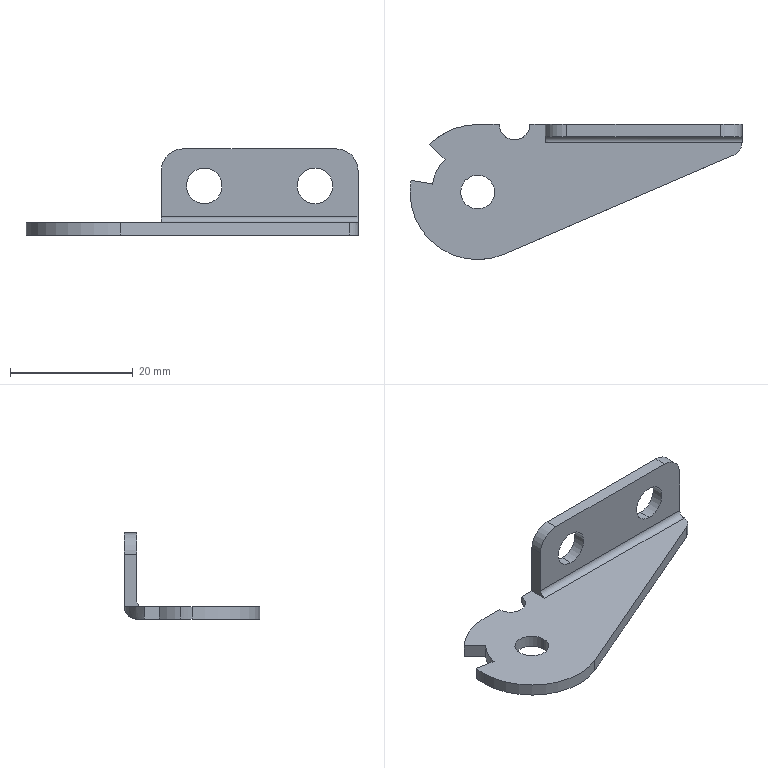Component | SolidWorks | MHPUS204-38-33-A-1_34-1 | 1 solid | 27 faces | box 54 x 22 x 14 mm | volume 2071 mm3 | cylinder 17 | plane 10 | commonest cylinder face diameters 5.8 x4 22 x3 5.5 x2 4 x2 7 x2 5 x1 4.4 x1 15 x1
STEP:
#1=CARTESIAN_POINT('',(20.81,-0.9055,1.98));
#2=VERTEX_POINT('',#1);
#3=CARTESIAN_POINT('',(20.594,-0.9055,1.98));
#4=VERTEX_POINT('',#3);
#5=CARTESIAN_POINT('',(20.702,-0.9055,1.98));
#6=DIRECTION('',(0.,0.,-1.));
#7=DIRECTION('',(-1.,0.,0.));
#8=AXIS2_PLACEMENT_3D('',#5,#6,#7);
#9=CIRCLE('',#8,0.1083);
#10=EDGE_CURVE('',#2,#4,#9,.T.);
#11=ORIENTED_EDGE('',*,*,#10,.F.);
#12=CARTESIAN_POINT('',(20.81,-0.9055,1.902));
#13=VERTEX_POINT('',#12);
#14=CARTESIAN_POINT('',(20.81,-0.9055,1.902));
#15=DIRECTION('',(0.,0.,-1.));
#16=VECTOR('',#15,39.37);
#17=LINE('',#14,#16);
#18=EDGE_CURVE('',#2,#13,#17,.T.);
#19=ORIENTED_EDGE('',*,*,#18,.T.);
#20=CARTESIAN_POINT('',(20.594,-0.9055,1.902));
#21=VERTEX_POINT('',#20);
#22=CARTESIAN_POINT('',(20.702,-0.9055,1.902));
#23=DIRECTION('',(0.,0.,-1.));
#24=DIRECTION('',(-1.,0.,0.));
#25=AXIS2_PLACEMENT_3D('',#22,#23,#24);
#26=CIRCLE('',#25,0.1083);
#27=EDGE_CURVE('',#13,#21,#26,.T.);
#28=ORIENTED_EDGE('',*,*,#27,.T.);
#29=CARTESIAN_POINT('',(20.594,-0.9055,1.902));
#30=DIRECTION('',(0.,0.,-1.));
#31=VECTOR('',#30,39.37);
#32=LINE('',#29,#31);
#33=EDGE_CURVE('',#4,#21,#32,.T.);
#34=ORIENTED_EDGE('',*,*,#33,.F.);
#35=EDGE_LOOP('',(#11,#19,#28,#34));
#36=FACE_OUTER_BOUND('',#35,.T.);
#37=CARTESIAN_POINT('',(20.702,-0.9055,1.902));
#38=DIRECTION('',(0.,0.,-1.));
#39=DIRECTION('',(-1.,0.,0.));
#40=AXIS2_PLACEMENT_3D('',#37,#38,#39);
#41=CYLINDRICAL_SURFACE('',#40,0.1083);
#42=ADVANCED_FACE('',(#36),#41,.F.);
#43=CARTESIAN_POINT('',(20.874,-1.303,1.98));
#44=VERTEX_POINT('',#43);
#45=CARTESIAN_POINT('',(20.269,-0.9055,1.98));
#46=VERTEX_POINT('',#45);
#47=CARTESIAN_POINT('',(20.702,-0.9055,1.98));
#48=DIRECTION('',(0.,0.,-1.));
#49=DIRECTION('',(-1.,0.,0.));
#50=AXIS2_PLACEMENT_3D('',#47,#48,#49);
#51=CIRCLE('',#50,0.4331);
#52=EDGE_CURVE('',#44,#46,#51,.T.);
#53=ORIENTED_EDGE('',*,*,#52,.T.);
#54=CARTESIAN_POINT('',(20.269,-0.9055,1.902));
#55=VERTEX_POINT('',#54);
#56=CARTESIAN_POINT('',(20.269,-0.9055,1.902));
#57=DIRECTION('',(0.,0.,-1.));
#58=VECTOR('',#57,39.37);
#59=LINE('',#56,#58);
#60=EDGE_CURVE('',#46,#55,#59,.T.);
#61=ORIENTED_EDGE('',*,*,#60,.T.);
#62=CARTESIAN_POINT('',(20.874,-1.303,1.902));
#63=VERTEX_POINT('',#62);
#64=CARTESIAN_POINT('',(20.702,-0.9055,1.902));
#65=DIRECTION('',(0.,0.,1.));
#66=DIRECTION('',(-1.,0.,0.));
#67=AXIS2_PLACEMENT_3D('',#64,#65,#66);
#68=CIRCLE('',#67,0.4331);
#69=EDGE_CURVE('',#55,#63,#68,.T.);
#70=ORIENTED_EDGE('',*,*,#69,.T.);
#71=CARTESIAN_POINT('',(20.874,-1.303,1.902));
#72=DIRECTION('',(0.,0.,-1.));
#73=VECTOR('',#72,39.37);
#74=LINE('',#71,#73);
#75=EDGE_CURVE('',#44,#63,#74,.T.);
#76=ORIENTED_EDGE('',*,*,#75,.F.);
#77=EDGE_LOOP('',(#53,#61,#70,#76));
#78=FACE_OUTER_BOUND('',#77,.T.);
#79=CARTESIAN_POINT('',(20.702,-0.9055,1.902));
#80=DIRECTION('',(0.,0.,-1.));
#81=DIRECTION('',(-1.,0.,0.));
#82=AXIS2_PLACEMENT_3D('',#79,#80,#81);
#83=CYLINDRICAL_SURFACE('',#82,0.4331);
#84=ADVANCED_FACE('',(#78),#83,.T.);
#85=CARTESIAN_POINT('',(21.411,-0.5512,2.331));
#86=VERTEX_POINT('',#85);
#87=CARTESIAN_POINT('',(21.411,-0.5512,2.102));
#88=VERTEX_POINT('',#87);
#89=CARTESIAN_POINT('',(21.411,-0.5512,2.217));
#90=DIRECTION('',(0.,-1.,0.));
#91=DIRECTION('',(0.,0.,1.));
#92=AXIS2_PLACEMENT_3D('',#89,#90,#91);
#93=CIRCLE('',#92,0.1142);
#94=EDGE_CURVE('',#86,#88,#93,.T.);
#95=ORIENTED_EDGE('',*,*,#94,.T.);
#96=CARTESIAN_POINT('',(21.411,-0.4724,2.102));
#97=VERTEX_POINT('',#96);
#98=CARTESIAN_POINT('',(21.411,-0.3937,2.102));
#99=DIRECTION('',(0.,1.,0.));
#100=VECTOR('',#99,39.37);
#101=LINE('',#98,#100);
#102=EDGE_CURVE('',#88,#97,#101,.T.);
#103=ORIENTED_EDGE('',*,*,#102,.T.);
#104=CARTESIAN_POINT('',(21.411,-0.4724,2.331));
#105=VERTEX_POINT('',#104);
#106=CARTESIAN_POINT('',(21.411,-0.4724,2.217));
#107=DIRECTION('',(0.,-1.,0.));
#108=DIRECTION('',(0.,0.,1.));
#109=AXIS2_PLACEMENT_3D('',#106,#107,#108);
#110=CIRCLE('',#109,0.1142);
#111=EDGE_CURVE('',#105,#97,#110,.T.);
#112=ORIENTED_EDGE('',*,*,#111,.F.);
#113=CARTESIAN_POINT('',(21.411,-0.3937,2.331));
#114=DIRECTION('',(0.,1.,0.));
#115=VECTOR('',#114,39.37);
#116=LINE('',#113,#115);
#117=EDGE_CURVE('',#86,#105,#116,.T.);
#118=ORIENTED_EDGE('',*,*,#117,.F.);
#119=EDGE_LOOP('',(#95,#103,#112,#118));
#120=FACE_OUTER_BOUND('',#119,.T.);
#121=CARTESIAN_POINT('',(21.411,-0.3937,2.217));
#122=DIRECTION('',(0.,1.,0.));
#123=DIRECTION('',(0.,0.,1.));
#124=AXIS2_PLACEMENT_3D('',#121,#122,#123);
#125=CYLINDRICAL_SURFACE('',#124,0.1142);
#126=ADVANCED_FACE('',(#120),#125,.F.);
#127=CARTESIAN_POINT('',(22.119,-0.5512,2.331));
#128=VERTEX_POINT('',#127);
#129=CARTESIAN_POINT('',(22.119,-0.5512,2.102));
#130=VERTEX_POINT('',#129);
#131=CARTESIAN_POINT('',(22.119,-0.5512,2.217));
#132=DIRECTION('',(0.,-1.,0.));
#133=DIRECTION('',(0.,0.,1.));
#134=AXIS2_PLACEMENT_3D('',#131,#132,#133);
#135=CIRCLE('',#134,0.1142);
#136=EDGE_CURVE('',#128,#130,#135,.T.);
#137=ORIENTED_EDGE('',*,*,#136,.T.);
#138=CARTESIAN_POINT('',(22.119,-0.4724,2.102));
#139=VERTEX_POINT('',#138);
#140=CARTESIAN_POINT('',(22.119,-0.3937,2.102));
#141=DIRECTION('',(0.,1.,0.));
#142=VECTOR('',#141,39.37);
#143=LINE('',#140,#142);
#144=EDGE_CURVE('',#130,#139,#143,.T.);
#145=ORIENTED_EDGE('',*,*,#144,.T.);
#146=CARTESIAN_POINT('',(22.119,-0.4724,2.331));
#147=VERTEX_POINT('',#146);
#148=CARTESIAN_POINT('',(22.119,-0.4724,2.217));
#149=DIRECTION('',(0.,-1.,0.));
#150=DIRECTION('',(0.,0.,1.));
#151=AXIS2_PLACEMENT_3D('',#148,#149,#150);
#152=CIRCLE('',#151,0.1142);
#153=EDGE_CURVE('',#147,#139,#152,.T.);
#154=ORIENTED_EDGE('',*,*,#153,.F.);
#155=CARTESIAN_POINT('',(22.119,-0.3937,2.331));
#156=DIRECTION('',(0.,1.,0.));
#157=VECTOR('',#156,39.37);
#158=LINE('',#155,#157);
#159=EDGE_CURVE('',#128,#147,#158,.T.);
#160=ORIENTED_EDGE('',*,*,#159,.F.);
#161=EDGE_LOOP('',(#137,#145,#154,#160));
#162=FACE_OUTER_BOUND('',#161,.T.);
#163=CARTESIAN_POINT('',(22.119,-0.3937,2.217));
#164=DIRECTION('',(0.,1.,0.));
#165=DIRECTION('',(0.,0.,1.));
#166=AXIS2_PLACEMENT_3D('',#163,#164,#165);
#167=CYLINDRICAL_SURFACE('',#166,0.1142);
#168=ADVANCED_FACE('',(#162),#167,.F.);
#169=CARTESIAN_POINT('',(20.702,-0.9055,1.902));
#170=DIRECTION('',(0.,0.,-1.));
#171=DIRECTION('',(-1.,0.,0.));
#172=AXIS2_PLACEMENT_3D('',#169,#170,#171);
#173=CIRCLE('',#172,0.1083);
#174=EDGE_CURVE('',#21,#13,#173,.T.);
#175=ORIENTED_EDGE('',*,*,#174,.F.);
#176=ORIENTED_EDGE('',*,*,#27,.F.);
#177=EDGE_LOOP('',(#175,#176));
#178=FACE_BOUND('',#177,.T.);
#179=CARTESIAN_POINT('',(22.395,-0.5512,1.902));
#180=VERTEX_POINT('',#179);
#181=CARTESIAN_POINT('',(20.997,-0.5512,1.902));
#182=VERTEX_POINT('',#181);
#183=CARTESIAN_POINT('',(20.702,-0.5512,1.902));
#184=DIRECTION('',(-1.,0.,0.));
#185=VECTOR('',#184,39.37);
#186=LINE('',#183,#185);
#187=EDGE_CURVE('',#180,#182,#186,.T.);
#188=ORIENTED_EDGE('',*,*,#187,.F.);
#189=CARTESIAN_POINT('',(22.395,-0.5887,1.902));
#190=VERTEX_POINT('',#189);
#191=CARTESIAN_POINT('',(22.395,-0.4724,1.902));
#192=DIRECTION('',(0.,1.,0.));
#193=VECTOR('',#192,39.37);
#194=LINE('',#191,#193);
#195=EDGE_CURVE('',#190,#180,#194,.T.);
#196=ORIENTED_EDGE('',*,*,#195,.F.);
#197=CARTESIAN_POINT('',(22.343,-0.6683,1.902));
#198=VERTEX_POINT('',#197);
#199=CARTESIAN_POINT('',(22.308,-0.5887,1.902));
#200=DIRECTION('',(0.,0.,1.));
#201=DIRECTION('',(-1.,-0.,0.));
#202=AXIS2_PLACEMENT_3D('',#199,#200,#201);
#203=CIRCLE('',#202,0.08661);
#204=EDGE_CURVE('',#198,#190,#203,.T.);
#205=ORIENTED_EDGE('',*,*,#204,.F.);
#206=CARTESIAN_POINT('',(20.874,-1.303,1.902));
#207=DIRECTION('',(0.9179,0.3967,0.));
#208=VECTOR('',#207,39.37);
#209=LINE('',#206,#208);
#210=EDGE_CURVE('',#63,#198,#209,.T.);
#211=ORIENTED_EDGE('',*,*,#210,.F.);
#212=ORIENTED_EDGE('',*,*,#69,.F.);
#213=CARTESIAN_POINT('',(20.276,-0.8303,1.902));
#214=VERTEX_POINT('',#213);
#215=CARTESIAN_POINT('',(20.702,-0.9055,1.902));
#216=DIRECTION('',(0.,0.,1.));
#217=DIRECTION('',(-1.,0.,0.));
#218=AXIS2_PLACEMENT_3D('',#215,#216,#217);
#219=CIRCLE('',#218,0.4331);
#220=EDGE_CURVE('',#214,#55,#219,.T.);
#221=ORIENTED_EDGE('',*,*,#220,.F.);
#222=CARTESIAN_POINT('',(20.411,-0.8542,1.902));
#223=VERTEX_POINT('',#222);
#224=CARTESIAN_POINT('',(20.411,-0.8542,1.902));
#225=DIRECTION('',(-0.9848,0.1736,0.));
#226=VECTOR('',#225,39.37);
#227=LINE('',#224,#226);
#228=EDGE_CURVE('',#223,#214,#227,.T.);
#229=ORIENTED_EDGE('',*,*,#228,.F.);
#230=CARTESIAN_POINT('',(20.493,-0.6967,1.902));
#231=VERTEX_POINT('',#230);
#232=CARTESIAN_POINT('',(20.702,-0.9055,1.902));
#233=DIRECTION('',(0.,0.,1.));
#234=DIRECTION('',(-1.,-0.,0.));
#235=AXIS2_PLACEMENT_3D('',#232,#233,#234);
#236=CIRCLE('',#235,0.2953);
#237=EDGE_CURVE('',#231,#223,#236,.T.);
#238=ORIENTED_EDGE('',*,*,#237,.F.);
#239=CARTESIAN_POINT('',(20.396,-0.5993,1.902));
#240=VERTEX_POINT('',#239);
#241=CARTESIAN_POINT('',(20.396,-0.5993,1.902));
#242=DIRECTION('',(0.7071,-0.7071,0.));
#243=VECTOR('',#242,39.37);
#244=LINE('',#241,#243);
#245=EDGE_CURVE('',#240,#231,#244,.T.);
#246=ORIENTED_EDGE('',*,*,#245,.F.);
#247=CARTESIAN_POINT('',(20.453,-0.5512,1.902));
#248=VERTEX_POINT('',#247);
#249=CARTESIAN_POINT('',(20.702,-0.9055,1.902));
#250=DIRECTION('',(0.,0.,1.));
#251=DIRECTION('',(-1.,-0.,0.));
#252=AXIS2_PLACEMENT_3D('',#249,#250,#251);
#253=CIRCLE('',#252,0.4331);
#254=EDGE_CURVE('',#248,#240,#253,.T.);
#255=ORIENTED_EDGE('',*,*,#254,.F.);
#256=CARTESIAN_POINT('',(20.879,-0.5512,1.902));
#257=VERTEX_POINT('',#256);
#258=CARTESIAN_POINT('',(20.702,-0.5512,1.902));
#259=DIRECTION('',(-1.,0.,0.));
#260=VECTOR('',#259,39.37);
#261=LINE('',#258,#260);
#262=EDGE_CURVE('',#257,#248,#261,.T.);
#263=ORIENTED_EDGE('',*,*,#262,.F.);
#264=CARTESIAN_POINT('',(20.938,-0.4724,1.902));
#265=DIRECTION('',(0.,0.,-1.));
#266=DIRECTION('',(-1.,0.,0.));
#267=AXIS2_PLACEMENT_3D('',#264,#265,#266);
#268=CIRCLE('',#267,0.09843);
#269=EDGE_CURVE('',#182,#257,#268,.T.);
#270=ORIENTED_EDGE('',*,*,#269,.F.);
#271=EDGE_LOOP('',(#188,#196,#205,#211,#212,#221,#229,#238,#246,#255,#263,#270));
#272=FACE_OUTER_BOUND('',#271,.T.);
#273=CARTESIAN_POINT('',(20.702,-1.339,1.902));
#274=DIRECTION('',(0.,0.,1.));
#275=DIRECTION('',(1.,0.,0.));
#276=AXIS2_PLACEMENT_3D('',#273,#274,#275);
#277=PLANE('',#276);
#278=ADVANCED_FACE('',(#178,#272),#277,.F.);
#279=ORIENTED_EDGE('',*,*,#18,.F.);
#280=CARTESIAN_POINT('',(20.702,-0.9055,1.98));
#281=DIRECTION('',(0.,0.,-1.));
#282=DIRECTION('',(-1.,0.,0.));
#283=AXIS2_PLACEMENT_3D('',#280,#281,#282);
#284=CIRCLE('',#283,0.1083);
#285=EDGE_CURVE('',#4,#2,#284,.T.);
#286=ORIENTED_EDGE('',*,*,#285,.F.);
#287=ORIENTED_EDGE('',*,*,#33,.T.);
#288=ORIENTED_EDGE('',*,*,#174,.T.);
#289=EDGE_LOOP('',(#279,#286,#287,#288));
#290=FACE_OUTER_BOUND('',#289,.T.);
#291=CARTESIAN_POINT('',(20.702,-0.9055,1.902));
#292=DIRECTION('',(0.,0.,-1.));
#293=DIRECTION('',(-1.,0.,0.));
#294=AXIS2_PLACEMENT_3D('',#291,#292,#293);
#295=CYLINDRICAL_SURFACE('',#294,0.1083);
#296=ADVANCED_FACE('',(#290),#295,.F.);
#297=CARTESIAN_POINT('',(21.037,-0.4724,1.98));
#298=VERTEX_POINT('',#297);
#299=CARTESIAN_POINT('',(20.84,-0.4724,1.98));
#300=VERTEX_POINT('',#299);
#301=CARTESIAN_POINT('',(20.938,-0.4724,1.98));
#302=DIRECTION('',(0.,0.,-1.));
#303=DIRECTION('',(-1.,0.,0.));
#304=AXIS2_PLACEMENT_3D('',#301,#302,#303);
#305=CIRCLE('',#304,0.09843);
#306=EDGE_CURVE('',#298,#300,#305,.T.);
#307=ORIENTED_EDGE('',*,*,#306,.F.);
#308=CARTESIAN_POINT('',(20.997,-0.5512,1.902));
#309=CARTESIAN_POINT('',(21.002,-0.5478,1.902));
#310=CARTESIAN_POINT('',(21.006,-0.544,1.902));
#311=CARTESIAN_POINT('',(21.014,-0.5359,1.903));
#312=CARTESIAN_POINT('',(21.017,-0.5314,1.904));
#313=CARTESIAN_POINT('',(21.023,-0.5224,1.907));
#314=CARTESIAN_POINT('',(21.026,-0.5177,1.909));
#315=CARTESIAN_POINT('',(21.03,-0.5085,1.914));
#316=CARTESIAN_POINT('',(21.032,-0.504,1.917));
#317=CARTESIAN_POINT('',(21.034,-0.4957,1.924));
#318=CARTESIAN_POINT('',(21.035,-0.4917,1.928));
#319=CARTESIAN_POINT('',(21.036,-0.485,1.937));
#320=CARTESIAN_POINT('',(21.036,-0.482,1.942));
#321=CARTESIAN_POINT('',(21.037,-0.4773,1.953));
#322=CARTESIAN_POINT('',(21.037,-0.4755,1.958));
#323=CARTESIAN_POINT('',(21.037,-0.4731,1.969));
#324=CARTESIAN_POINT('',(21.037,-0.4724,1.975));
#325=CARTESIAN_POINT('',(21.037,-0.4724,1.98));
#326=B_SPLINE_CURVE_WITH_KNOTS('',3,(#308,#309,#310,#311,#312,#313,#314,#315,#316,#317,#318,#319,#320,#321,#322,#323,#324,#325),.UNSPECIFIED.,.F.,.F.,(4,2,2,2,2,2,2,2,4),(0.,0.0004287,0.0008574,0.001286,0.001715,0.002144,0.002572,0.003001,0.00343),.UNSPECIFIED.);
#327=EDGE_CURVE('',#182,#298,#326,.T.);
#328=ORIENTED_EDGE('',*,*,#327,.F.);
#329=ORIENTED_EDGE('',*,*,#269,.T.);
#330=CARTESIAN_POINT('',(20.84,-0.4724,1.98));
#331=CARTESIAN_POINT('',(20.84,-0.4724,1.975));
#332=CARTESIAN_POINT('',(20.84,-0.4731,1.969));
#333=CARTESIAN_POINT('',(20.84,-0.4755,1.958));
#334=CARTESIAN_POINT('',(20.84,-0.4773,1.953));
#335=CARTESIAN_POINT('',(20.84,-0.482,1.942));
#336=CARTESIAN_POINT('',(20.841,-0.4849,1.937));
#337=CARTESIAN_POINT('',(20.842,-0.4917,1.928));
#338=CARTESIAN_POINT('',(20.843,-0.4955,1.924));
#339=CARTESIAN_POINT('',(20.845,-0.5038,1.917));
#340=CARTESIAN_POINT('',(20.847,-0.5084,1.914));
#341=CARTESIAN_POINT('',(20.851,-0.5175,1.909));
#342=CARTESIAN_POINT('',(20.853,-0.5222,1.907));
#343=CARTESIAN_POINT('',(20.862,-0.5359,1.902));
#344=CARTESIAN_POINT('',(20.87,-0.5443,1.902));
#345=CARTESIAN_POINT('',(20.879,-0.5512,1.902));
#346=B_SPLINE_CURVE_WITH_KNOTS('',3,(#330,#331,#332,#333,#334,#335,#336,#337,#338,#339,#340,#341,#342,#343,#344,#345),.UNSPECIFIED.,.F.,.F.,(4,2,2,2,2,2,2,4),(0.,0.0004284,0.0008569,0.001285,0.001714,0.002142,0.002571,0.003428),.UNSPECIFIED.);
#347=EDGE_CURVE('',#300,#257,#346,.T.);
#348=ORIENTED_EDGE('',*,*,#347,.F.);
#349=EDGE_LOOP('',(#307,#328,#329,#348));
#350=FACE_OUTER_BOUND('',#349,.T.);
#351=CARTESIAN_POINT('',(20.938,-0.4724,1.902));
#352=DIRECTION('',(0.,0.,-1.));
#353=DIRECTION('',(-1.,0.,0.));
#354=AXIS2_PLACEMENT_3D('',#351,#352,#353);
#355=CYLINDRICAL_SURFACE('',#354,0.09843);
#356=ADVANCED_FACE('',(#350),#355,.F.);
#357=CARTESIAN_POINT('',(22.395,-0.4724,1.98));
#358=VERTEX_POINT('',#357);
#359=CARTESIAN_POINT('',(22.395,-0.5512,1.98));
#360=DIRECTION('',(-1.,0.,0.));
#361=DIRECTION('',(0.,0.,-1.));
#362=AXIS2_PLACEMENT_3D('',#359,#360,#361);
#363=CIRCLE('',#362,0.07874);
#364=EDGE_CURVE('',#358,#180,#363,.T.);
#365=ORIENTED_EDGE('',*,*,#364,.T.);
#366=ORIENTED_EDGE('',*,*,#187,.T.);
#367=ORIENTED_EDGE('',*,*,#327,.T.);
#368=CARTESIAN_POINT('',(21.135,-0.4724,1.98));
#369=VERTEX_POINT('',#368);
#370=CARTESIAN_POINT('',(23.261,-0.4724,1.98));
#371=DIRECTION('',(1.,0.,0.));
#372=VECTOR('',#371,39.37);
#373=LINE('',#370,#372);
#374=EDGE_CURVE('',#298,#369,#373,.T.);
#375=ORIENTED_EDGE('',*,*,#374,.T.);
#376=CARTESIAN_POINT('',(23.261,-0.4724,1.98));
#377=DIRECTION('',(1.,0.,0.));
#378=VECTOR('',#377,39.37);
#379=LINE('',#376,#378);
#380=EDGE_CURVE('',#369,#358,#379,.T.);
#381=ORIENTED_EDGE('',*,*,#380,.T.);
#382=EDGE_LOOP('',(#365,#366,#367,#375,#381));
#383=FACE_OUTER_BOUND('',#382,.T.);
#384=CARTESIAN_POINT('',(23.261,-0.5512,1.98));
#385=DIRECTION('',(1.,0.,0.));
#386=DIRECTION('',(0.,0.,-1.));
#387=AXIS2_PLACEMENT_3D('',#384,#385,#386);
#388=CYLINDRICAL_SURFACE('',#387,0.07874);
#389=ADVANCED_FACE('',(#383),#388,.T.);
#390=CARTESIAN_POINT('',(22.395,-0.5887,1.98));
#391=VERTEX_POINT('',#390);
#392=CARTESIAN_POINT('',(22.395,-0.5887,1.902));
#393=DIRECTION('',(0.,0.,1.));
#394=VECTOR('',#393,39.37);
#395=LINE('',#392,#394);
#396=EDGE_CURVE('',#190,#391,#395,.T.);
#397=ORIENTED_EDGE('',*,*,#396,.T.);
#398=CARTESIAN_POINT('',(22.395,-0.5906,1.98));
#399=VERTEX_POINT('',#398);
#400=CARTESIAN_POINT('',(22.395,-0.5887,1.98));
#401=CARTESIAN_POINT('',(22.395,-0.5893,1.98));
#402=CARTESIAN_POINT('',(22.395,-0.5899,1.98));
#403=CARTESIAN_POINT('',(22.395,-0.5906,1.98));
#404=B_SPLINE_CURVE_WITH_KNOTS('',3,(#400,#401,#402,#403),.UNSPECIFIED.,.F.,.F.,(4,4),(0.,0.0000459),.UNSPECIFIED.);
#405=EDGE_CURVE('',#391,#399,#404,.T.);
#406=ORIENTED_EDGE('',*,*,#405,.T.);
#407=CARTESIAN_POINT('',(22.343,-0.6683,1.98));
#408=VERTEX_POINT('',#407);
#409=CARTESIAN_POINT('',(22.308,-0.5887,1.98));
#410=DIRECTION('',(0.,0.,-1.));
#411=DIRECTION('',(-1.,0.,0.));
#412=AXIS2_PLACEMENT_3D('',#409,#410,#411);
#413=CIRCLE('',#412,0.08661);
#414=EDGE_CURVE('',#399,#408,#413,.T.);
#415=ORIENTED_EDGE('',*,*,#414,.T.);
#416=CARTESIAN_POINT('',(22.343,-0.6683,1.902));
#417=DIRECTION('',(0.,0.,-1.));
#418=VECTOR('',#417,39.37);
#419=LINE('',#416,#418);
#420=EDGE_CURVE('',#408,#198,#419,.T.);
#421=ORIENTED_EDGE('',*,*,#420,.T.);
#422=ORIENTED_EDGE('',*,*,#204,.T.);
#423=EDGE_LOOP('',(#397,#406,#415,#421,#422));
#424=FACE_OUTER_BOUND('',#423,.T.);
#425=CARTESIAN_POINT('',(22.308,-0.5887,1.902));
#426=DIRECTION('',(0.,0.,-1.));
#427=DIRECTION('',(-1.,0.,0.));
#428=AXIS2_PLACEMENT_3D('',#425,#426,#427);
#429=CYLINDRICAL_SURFACE('',#428,0.08661);
#430=ADVANCED_FACE('',(#424),#429,.T.);
#431=ORIENTED_EDGE('',*,*,#210,.T.);
#432=ORIENTED_EDGE('',*,*,#420,.F.);
#433=CARTESIAN_POINT('',(22.343,-0.6683,1.98));
#434=DIRECTION('',(-0.9179,-0.3967,0.));
#435=VECTOR('',#434,39.37);
#436=LINE('',#433,#435);
#437=EDGE_CURVE('',#408,#44,#436,.T.);
#438=ORIENTED_EDGE('',*,*,#437,.T.);
#439=ORIENTED_EDGE('',*,*,#75,.T.);
#440=EDGE_LOOP('',(#431,#432,#438,#439));
#441=FACE_OUTER_BOUND('',#440,.T.);
#442=CARTESIAN_POINT('',(22.343,-0.6683,1.902));
#443=DIRECTION('',(0.3967,-0.9179,0.));
#444=DIRECTION('',(0.9179,0.3967,0.));
#445=AXIS2_PLACEMENT_3D('',#442,#443,#444);
#446=PLANE('',#445);
#447=ADVANCED_FACE('',(#441),#446,.T.);
#448=ORIENTED_EDGE('',*,*,#60,.F.);
#449=CARTESIAN_POINT('',(20.276,-0.8303,1.98));
#450=VERTEX_POINT('',#449);
#451=CARTESIAN_POINT('',(20.702,-0.9055,1.98));
#452=DIRECTION('',(0.,0.,-1.));
#453=DIRECTION('',(-1.,0.,0.));
#454=AXIS2_PLACEMENT_3D('',#451,#452,#453);
#455=CIRCLE('',#454,0.4331);
#456=EDGE_CURVE('',#46,#450,#455,.T.);
#457=ORIENTED_EDGE('',*,*,#456,.T.);
#458=CARTESIAN_POINT('',(20.276,-0.8303,1.902));
#459=DIRECTION('',(0.,0.,-1.));
#460=VECTOR('',#459,39.37);
#461=LINE('',#458,#460);
#462=EDGE_CURVE('',#450,#214,#461,.T.);
#463=ORIENTED_EDGE('',*,*,#462,.T.);
#464=ORIENTED_EDGE('',*,*,#220,.T.);
#465=EDGE_LOOP('',(#448,#457,#463,#464));
#466=FACE_OUTER_BOUND('',#465,.T.);
#467=CARTESIAN_POINT('',(20.702,-0.9055,1.902));
#468=DIRECTION('',(0.,0.,-1.));
#469=DIRECTION('',(-1.,0.,0.));
#470=AXIS2_PLACEMENT_3D('',#467,#468,#469);
#471=CYLINDRICAL_SURFACE('',#470,0.4331);
#472=ADVANCED_FACE('',(#466),#471,.T.);
#473=ORIENTED_EDGE('',*,*,#228,.T.);
#474=ORIENTED_EDGE('',*,*,#462,.F.);
#475=CARTESIAN_POINT('',(20.411,-0.8542,1.98));
#476=VERTEX_POINT('',#475);
#477=CARTESIAN_POINT('',(20.276,-0.8303,1.98));
#478=DIRECTION('',(0.9848,-0.1736,0.));
#479=VECTOR('',#478,39.37);
#480=LINE('',#477,#479);
#481=EDGE_CURVE('',#450,#476,#480,.T.);
#482=ORIENTED_EDGE('',*,*,#481,.T.);
#483=CARTESIAN_POINT('',(20.411,-0.8542,1.902));
#484=DIRECTION('',(0.,0.,-1.));
#485=VECTOR('',#484,39.37);
#486=LINE('',#483,#485);
#487=EDGE_CURVE('',#476,#223,#486,.T.);
#488=ORIENTED_EDGE('',*,*,#487,.T.);
#489=EDGE_LOOP('',(#473,#474,#482,#488));
#490=FACE_OUTER_BOUND('',#489,.T.);
#491=CARTESIAN_POINT('',(20.276,-0.8303,1.902));
#492=DIRECTION('',(0.1736,0.9848,0.));
#493=DIRECTION('',(-0.9848,0.1736,0.));
#494=AXIS2_PLACEMENT_3D('',#491,#492,#493);
#495=PLANE('',#494);
#496=ADVANCED_FACE('',(#490),#495,.T.);
#497=ORIENTED_EDGE('',*,*,#237,.T.);
#498=ORIENTED_EDGE('',*,*,#487,.F.);
#499=CARTESIAN_POINT('',(20.493,-0.6967,1.98));
#500=VERTEX_POINT('',#499);
#501=CARTESIAN_POINT('',(20.702,-0.9055,1.98));
#502=DIRECTION('',(0.,0.,-1.));
#503=DIRECTION('',(-1.,0.,0.));
#504=AXIS2_PLACEMENT_3D('',#501,#502,#503);
#505=CIRCLE('',#504,0.2953);
#506=EDGE_CURVE('',#476,#500,#505,.T.);
#507=ORIENTED_EDGE('',*,*,#506,.T.);
#508=CARTESIAN_POINT('',(20.493,-0.6967,1.902));
#509=DIRECTION('',(0.,0.,-1.));
#510=VECTOR('',#509,39.37);
#511=LINE('',#508,#510);
#512=EDGE_CURVE('',#500,#231,#511,.T.);
#513=ORIENTED_EDGE('',*,*,#512,.T.);
#514=EDGE_LOOP('',(#497,#498,#507,#513));
#515=FACE_OUTER_BOUND('',#514,.T.);
#516=CARTESIAN_POINT('',(20.702,-0.9055,1.902));
#517=DIRECTION('',(0.,0.,-1.));
#518=DIRECTION('',(-1.,0.,0.));
#519=AXIS2_PLACEMENT_3D('',#516,#517,#518);
#520=CYLINDRICAL_SURFACE('',#519,0.2953);
#521=ADVANCED_FACE('',(#515),#520,.T.);
#522=ORIENTED_EDGE('',*,*,#245,.T.);
#523=ORIENTED_EDGE('',*,*,#512,.F.);
#524=CARTESIAN_POINT('',(20.396,-0.5993,1.98));
#525=VERTEX_POINT('',#524);
#526=CARTESIAN_POINT('',(20.493,-0.6967,1.98));
#527=DIRECTION('',(-0.7071,0.7071,0.));
#528=VECTOR('',#527,39.37);
#529=LINE('',#526,#528);
#530=EDGE_CURVE('',#500,#525,#529,.T.);
#531=ORIENTED_EDGE('',*,*,#530,.T.);
#532=CARTESIAN_POINT('',(20.396,-0.5993,1.902));
#533=DIRECTION('',(0.,0.,-1.));
#534=VECTOR('',#533,39.37);
#535=LINE('',#532,#534);
#536=EDGE_CURVE('',#525,#240,#535,.T.);
#537=ORIENTED_EDGE('',*,*,#536,.T.);
#538=EDGE_LOOP('',(#522,#523,#531,#537));
#539=FACE_OUTER_BOUND('',#538,.T.);
#540=CARTESIAN_POINT('',(20.493,-0.6967,1.902));
#541=DIRECTION('',(-0.7071,-0.7071,0.));
#542=DIRECTION('',(0.7071,-0.7071,0.));
#543=AXIS2_PLACEMENT_3D('',#540,#541,#542);
#544=PLANE('',#543);
#545=ADVANCED_FACE('',(#539),#544,.T.);
#546=ORIENTED_EDGE('',*,*,#254,.T.);
#547=ORIENTED_EDGE('',*,*,#536,.F.);
#548=CARTESIAN_POINT('',(20.702,-0.4724,1.98));
#549=VERTEX_POINT('',#548);
#550=CARTESIAN_POINT('',(20.702,-0.9055,1.98));
#551=DIRECTION('',(0.,0.,-1.));
#552=DIRECTION('',(-1.,0.,0.));
#553=AXIS2_PLACEMENT_3D('',#550,#551,#552);
#554=CIRCLE('',#553,0.4331);
#555=EDGE_CURVE('',#525,#549,#554,.T.);
#556=ORIENTED_EDGE('',*,*,#555,.T.);
#557=CARTESIAN_POINT('',(20.702,-0.4724,1.98));
#558=CARTESIAN_POINT('',(20.697,-0.4724,1.978));
#559=CARTESIAN_POINT('',(20.691,-0.4725,1.976));
#560=CARTESIAN_POINT('',(20.681,-0.4729,1.971));
#561=CARTESIAN_POINT('',(20.675,-0.4732,1.969));
#562=CARTESIAN_POINT('',(20.659,-0.4744,1.962));
#563=CARTESIAN_POINT('',(20.649,-0.4756,1.958));
#564=CARTESIAN_POINT('',(20.617,-0.4803,1.945));
#565=CARTESIAN_POINT('',(20.596,-0.485,1.936));
#566=CARTESIAN_POINT('',(20.565,-0.4947,1.925));
#567=CARTESIAN_POINT('',(20.554,-0.4984,1.922));
#568=CARTESIAN_POINT('',(20.533,-0.5066,1.915));
#569=CARTESIAN_POINT('',(20.523,-0.5111,1.912));
#570=CARTESIAN_POINT('',(20.492,-0.526,1.905));
#571=CARTESIAN_POINT('',(20.472,-0.5378,1.902));
#572=CARTESIAN_POINT('',(20.453,-0.5512,1.902));
#573=B_SPLINE_CURVE_WITH_KNOTS('',3,(#557,#558,#559,#560,#561,#562,#563,#564,#565,#566,#567,#568,#569,#570,#571,#572),.UNSPECIFIED.,.F.,.F.,(4,2,2,2,2,2,2,4),(-0.00002098,0.0004178,0.0008566,0.001734,0.003489,0.004367,0.005244,0.006999),.UNSPECIFIED.);
#574=EDGE_CURVE('',#549,#248,#573,.T.);
#575=ORIENTED_EDGE('',*,*,#574,.T.);
#576=EDGE_LOOP('',(#546,#547,#556,#575));
#577=FACE_OUTER_BOUND('',#576,.T.);
#578=CARTESIAN_POINT('',(20.702,-0.9055,1.902));
#579=DIRECTION('',(0.,0.,-1.));
#580=DIRECTION('',(-1.,0.,0.));
#581=AXIS2_PLACEMENT_3D('',#578,#579,#580);
#582=CYLINDRICAL_SURFACE('',#581,0.4331);
#583=ADVANCED_FACE('',(#577),#582,.T.);
#584=ORIENTED_EDGE('',*,*,#574,.F.);
#585=CARTESIAN_POINT('',(23.261,-0.4724,1.98));
#586=DIRECTION('',(1.,0.,0.));
#587=VECTOR('',#586,39.37);
#588=LINE('',#585,#587);
#589=EDGE_CURVE('',#549,#300,#588,.T.);
#590=ORIENTED_EDGE('',*,*,#589,.T.);
#591=ORIENTED_EDGE('',*,*,#347,.T.);
#592=ORIENTED_EDGE('',*,*,#262,.T.);
#593=EDGE_LOOP('',(#584,#590,#591,#592));
#594=FACE_OUTER_BOUND('',#593,.T.);
#595=CARTESIAN_POINT('',(23.261,-0.5512,1.98));
#596=DIRECTION('',(1.,0.,0.));
#597=DIRECTION('',(0.,0.,-1.));
#598=AXIS2_PLACEMENT_3D('',#595,#596,#597);
#599=CYLINDRICAL_SURFACE('',#598,0.07874);
#600=ADVANCED_FACE('',(#594),#599,.T.);
#601=ORIENTED_EDGE('',*,*,#285,.T.);
#602=ORIENTED_EDGE('',*,*,#10,.T.);
#603=EDGE_LOOP('',(#601,#602));
#604=FACE_BOUND('',#603,.T.);
#605=ORIENTED_EDGE('',*,*,#589,.F.);
#606=ORIENTED_EDGE('',*,*,#555,.F.);
#607=ORIENTED_EDGE('',*,*,#530,.F.);
#608=ORIENTED_EDGE('',*,*,#506,.F.);
#609=ORIENTED_EDGE('',*,*,#481,.F.);
#610=ORIENTED_EDGE('',*,*,#456,.F.);
#611=ORIENTED_EDGE('',*,*,#52,.F.);
#612=ORIENTED_EDGE('',*,*,#437,.F.);
#613=ORIENTED_EDGE('',*,*,#414,.F.);
#614=CARTESIAN_POINT('',(21.135,-0.5906,1.98));
#615=VERTEX_POINT('',#614);
#616=CARTESIAN_POINT('',(23.261,-0.5906,1.98));
#617=DIRECTION('',(1.,0.,0.));
#618=VECTOR('',#617,39.37);
#619=LINE('',#616,#618);
#620=EDGE_CURVE('',#615,#399,#619,.T.);
#621=ORIENTED_EDGE('',*,*,#620,.F.);
#622=CARTESIAN_POINT('',(21.135,-1.339,1.98));
#623=DIRECTION('',(0.,-1.,0.));
#624=VECTOR('',#623,39.37);
#625=LINE('',#622,#624);
#626=EDGE_CURVE('',#369,#615,#625,.T.);
#627=ORIENTED_EDGE('',*,*,#626,.F.);
#628=ORIENTED_EDGE('',*,*,#374,.F.);
#629=ORIENTED_EDGE('',*,*,#306,.T.);
#630=EDGE_LOOP('',(#605,#606,#607,#608,#609,#610,#611,#612,#613,#621,#627,#628,#629));
#631=FACE_OUTER_BOUND('',#630,.T.);
#632=CARTESIAN_POINT('',(23.261,-1.339,1.98));
#633=DIRECTION('',(0.,0.,-1.));
#634=DIRECTION('',(-1.,0.,0.));
#635=AXIS2_PLACEMENT_3D('',#632,#633,#634);
#636=PLANE('',#635);
#637=ADVANCED_FACE('',(#604,#631),#636,.F.);
#638=ORIENTED_EDGE('',*,*,#364,.F.);
#639=CARTESIAN_POINT('',(22.395,-0.4724,2.315));
#640=VERTEX_POINT('',#639);
#641=CARTESIAN_POINT('',(22.395,-0.4724,1.902));
#642=DIRECTION('',(0.,0.,1.));
#643=VECTOR('',#642,39.37);
#644=LINE('',#641,#643);
#645=EDGE_CURVE('',#358,#640,#644,.T.);
#646=ORIENTED_EDGE('',*,*,#645,.T.);
#647=CARTESIAN_POINT('',(22.395,-0.5512,2.315));
#648=VERTEX_POINT('',#647);
#649=CARTESIAN_POINT('',(22.395,-0.4724,2.315));
#650=DIRECTION('',(0.,-1.,0.));
#651=VECTOR('',#650,39.37);
#652=LINE('',#649,#651);
#653=EDGE_CURVE('',#640,#648,#652,.T.);
#654=ORIENTED_EDGE('',*,*,#653,.T.);
#655=CARTESIAN_POINT('',(22.395,-0.5512,2.02));
#656=VERTEX_POINT('',#655);
#657=CARTESIAN_POINT('',(22.395,-0.5512,1.902));
#658=DIRECTION('',(0.,0.,-1.));
#659=VECTOR('',#658,39.37);
#660=LINE('',#657,#659);
#661=EDGE_CURVE('',#648,#656,#660,.T.);
#662=ORIENTED_EDGE('',*,*,#661,.T.);
#663=CARTESIAN_POINT('',(22.395,-0.5906,2.02));
#664=DIRECTION('',(-1.,0.,0.));
#665=DIRECTION('',(0.,0.,-1.));
#666=AXIS2_PLACEMENT_3D('',#663,#664,#665);
#667=CIRCLE('',#666,0.03937);
#668=EDGE_CURVE('',#656,#391,#667,.T.);
#669=ORIENTED_EDGE('',*,*,#668,.T.);
#670=ORIENTED_EDGE('',*,*,#396,.F.);
#671=ORIENTED_EDGE('',*,*,#195,.T.);
#672=EDGE_LOOP('',(#638,#646,#654,#662,#669,#670,#671));
#673=FACE_OUTER_BOUND('',#672,.T.);
#674=CARTESIAN_POINT('',(22.395,-0.4724,1.902));
#675=DIRECTION('',(1.,0.,0.));
#676=DIRECTION('',(0.,0.,-1.));
#677=AXIS2_PLACEMENT_3D('',#674,#675,#676);
#678=PLANE('',#677);
#679=ADVANCED_FACE('',(#673),#678,.T.);
#680=ORIENTED_EDGE('',*,*,#645,.F.);
#681=ORIENTED_EDGE('',*,*,#380,.F.);
#682=CARTESIAN_POINT('',(21.135,-0.4724,2.315));
#683=VERTEX_POINT('',#682);
#684=CARTESIAN_POINT('',(21.135,-0.4724,1.902));
#685=DIRECTION('',(0.,0.,1.));
#686=VECTOR('',#685,39.37);
#687=LINE('',#684,#686);
#688=EDGE_CURVE('',#369,#683,#687,.T.);
#689=ORIENTED_EDGE('',*,*,#688,.T.);
#690=CARTESIAN_POINT('',(21.273,-0.4724,2.453));
#691=VERTEX_POINT('',#690);
#692=CARTESIAN_POINT('',(21.273,-0.4724,2.315));
#693=DIRECTION('',(0.,1.,0.));
#694=DIRECTION('',(0.,0.,-1.));
#695=AXIS2_PLACEMENT_3D('',#692,#693,#694);
#696=CIRCLE('',#695,0.1378);
#697=EDGE_CURVE('',#683,#691,#696,.T.);
#698=ORIENTED_EDGE('',*,*,#697,.T.);
#699=CARTESIAN_POINT('',(22.257,-0.4724,2.453));
#700=VERTEX_POINT('',#699);
#701=CARTESIAN_POINT('',(20.702,-0.4724,2.453));
#702=DIRECTION('',(1.,0.,0.));
#703=VECTOR('',#702,39.37);
#704=LINE('',#701,#703);
#705=EDGE_CURVE('',#691,#700,#704,.T.);
#706=ORIENTED_EDGE('',*,*,#705,.T.);
#707=CARTESIAN_POINT('',(22.257,-0.4724,2.315));
#708=DIRECTION('',(0.,1.,0.));
#709=DIRECTION('',(0.,0.,-1.));
#710=AXIS2_PLACEMENT_3D('',#707,#708,#709);
#711=CIRCLE('',#710,0.1378);
#712=EDGE_CURVE('',#700,#640,#711,.T.);
#713=ORIENTED_EDGE('',*,*,#712,.T.);
#714=EDGE_LOOP('',(#680,#681,#689,#698,#706,#713));
#715=FACE_OUTER_BOUND('',#714,.T.);
#716=ORIENTED_EDGE('',*,*,#111,.T.);
#717=CARTESIAN_POINT('',(21.411,-0.4724,2.217));
#718=DIRECTION('',(0.,-1.,0.));
#719=DIRECTION('',(0.,0.,1.));
#720=AXIS2_PLACEMENT_3D('',#717,#718,#719);
#721=CIRCLE('',#720,0.1142);
#722=EDGE_CURVE('',#97,#105,#721,.T.);
#723=ORIENTED_EDGE('',*,*,#722,.T.);
#724=EDGE_LOOP('',(#716,#723));
#725=FACE_BOUND('',#724,.T.);
#726=ORIENTED_EDGE('',*,*,#153,.T.);
#727=CARTESIAN_POINT('',(22.119,-0.4724,2.217));
#728=DIRECTION('',(0.,-1.,0.));
#729=DIRECTION('',(0.,0.,1.));
#730=AXIS2_PLACEMENT_3D('',#727,#728,#729);
#731=CIRCLE('',#730,0.1142);
#732=EDGE_CURVE('',#139,#147,#731,.T.);
#733=ORIENTED_EDGE('',*,*,#732,.T.);
#734=EDGE_LOOP('',(#726,#733));
#735=FACE_BOUND('',#734,.T.);
#736=CARTESIAN_POINT('',(20.702,-0.4724,1.902));
#737=DIRECTION('',(0.,1.,0.));
#738=DIRECTION('',(0.,0.,1.));
#739=AXIS2_PLACEMENT_3D('',#736,#737,#738);
#740=PLANE('',#739);
#741=ADVANCED_FACE('',(#715,#725,#735),#740,.T.);
#742=ORIENTED_EDGE('',*,*,#620,.T.);
#743=ORIENTED_EDGE('',*,*,#405,.F.);
#744=ORIENTED_EDGE('',*,*,#668,.F.);
#745=CARTESIAN_POINT('',(21.135,-0.5512,2.02));
#746=VERTEX_POINT('',#745);
#747=CARTESIAN_POINT('',(23.261,-0.5512,2.02));
#748=DIRECTION('',(1.,0.,0.));
#749=VECTOR('',#748,39.37);
#750=LINE('',#747,#749);
#751=EDGE_CURVE('',#746,#656,#750,.T.);
#752=ORIENTED_EDGE('',*,*,#751,.F.);
#753=CARTESIAN_POINT('',(21.135,-0.5906,2.02));
#754=DIRECTION('',(1.,0.,0.));
#755=DIRECTION('',(0.,0.,-1.));
#756=AXIS2_PLACEMENT_3D('',#753,#754,#755);
#757=CIRCLE('',#756,0.03937);
#758=EDGE_CURVE('',#615,#746,#757,.T.);
#759=ORIENTED_EDGE('',*,*,#758,.F.);
#760=EDGE_LOOP('',(#742,#743,#744,#752,#759));
#761=FACE_OUTER_BOUND('',#760,.T.);
#762=CARTESIAN_POINT('',(23.261,-0.5906,2.02));
#763=DIRECTION('',(1.,0.,0.));
#764=DIRECTION('',(0.,0.,-1.));
#765=AXIS2_PLACEMENT_3D('',#762,#763,#764);
#766=CYLINDRICAL_SURFACE('',#765,0.03937);
#767=ADVANCED_FACE('',(#761),#766,.F.);
#768=CARTESIAN_POINT('',(21.135,-0.5512,2.315));
#769=VERTEX_POINT('',#768);
#770=CARTESIAN_POINT('',(21.135,-1.339,2.315));
#771=DIRECTION('',(0.,-1.,0.));
#772=VECTOR('',#771,39.37);
#773=LINE('',#770,#772);
#774=EDGE_CURVE('',#683,#769,#773,.T.);
#775=ORIENTED_EDGE('',*,*,#774,.F.);
#776=ORIENTED_EDGE('',*,*,#688,.F.);
#777=ORIENTED_EDGE('',*,*,#626,.T.);
#778=ORIENTED_EDGE('',*,*,#758,.T.);
#779=CARTESIAN_POINT('',(21.135,-0.5512,1.98));
#780=DIRECTION('',(0.,0.,-1.));
#781=VECTOR('',#780,39.37);
#782=LINE('',#779,#781);
#783=EDGE_CURVE('',#769,#746,#782,.T.);
#784=ORIENTED_EDGE('',*,*,#783,.F.);
#785=EDGE_LOOP('',(#775,#776,#777,#778,#784));
#786=FACE_OUTER_BOUND('',#785,.T.);
#787=CARTESIAN_POINT('',(21.135,-1.339,1.98));
#788=DIRECTION('',(1.,0.,0.));
#789=DIRECTION('',(0.,0.,-1.));
#790=AXIS2_PLACEMENT_3D('',#787,#788,#789);
#791=PLANE('',#790);
#792=ADVANCED_FACE('',(#786),#791,.F.);
#793=ORIENTED_EDGE('',*,*,#751,.T.);
#794=ORIENTED_EDGE('',*,*,#661,.F.);
#795=CARTESIAN_POINT('',(22.257,-0.5512,2.453));
#796=VERTEX_POINT('',#795);
#797=CARTESIAN_POINT('',(22.257,-0.5512,2.315));
#798=DIRECTION('',(0.,1.,0.));
#799=DIRECTION('',(0.,0.,-1.));
#800=AXIS2_PLACEMENT_3D('',#797,#798,#799);
#801=CIRCLE('',#800,0.1378);
#802=EDGE_CURVE('',#796,#648,#801,.T.);
#803=ORIENTED_EDGE('',*,*,#802,.F.);
#804=CARTESIAN_POINT('',(21.273,-0.5512,2.453));
#805=VERTEX_POINT('',#804);
#806=CARTESIAN_POINT('',(23.261,-0.5512,2.453));
#807=DIRECTION('',(1.,0.,0.));
#808=VECTOR('',#807,39.37);
#809=LINE('',#806,#808);
#810=EDGE_CURVE('',#805,#796,#809,.T.);
#811=ORIENTED_EDGE('',*,*,#810,.F.);
#812=CARTESIAN_POINT('',(21.273,-0.5512,2.315));
#813=DIRECTION('',(0.,1.,0.));
#814=DIRECTION('',(0.,0.,-1.));
#815=AXIS2_PLACEMENT_3D('',#812,#813,#814);
#816=CIRCLE('',#815,0.1378);
#817=EDGE_CURVE('',#769,#805,#816,.T.);
#818=ORIENTED_EDGE('',*,*,#817,.F.);
#819=ORIENTED_EDGE('',*,*,#783,.T.);
#820=EDGE_LOOP('',(#793,#794,#803,#811,#818,#819));
#821=FACE_OUTER_BOUND('',#820,.T.);
#822=ORIENTED_EDGE('',*,*,#94,.F.);
#823=CARTESIAN_POINT('',(21.411,-0.5512,2.217));
#824=DIRECTION('',(0.,-1.,0.));
#825=DIRECTION('',(0.,0.,1.));
#826=AXIS2_PLACEMENT_3D('',#823,#824,#825);
#827=CIRCLE('',#826,0.1142);
#828=EDGE_CURVE('',#88,#86,#827,.T.);
#829=ORIENTED_EDGE('',*,*,#828,.F.);
#830=EDGE_LOOP('',(#822,#829));
#831=FACE_BOUND('',#830,.T.);
#832=ORIENTED_EDGE('',*,*,#136,.F.);
#833=CARTESIAN_POINT('',(22.119,-0.5512,2.217));
#834=DIRECTION('',(0.,-1.,0.));
#835=DIRECTION('',(0.,0.,1.));
#836=AXIS2_PLACEMENT_3D('',#833,#834,#835);
#837=CIRCLE('',#836,0.1142);
#838=EDGE_CURVE('',#130,#128,#837,.T.);
#839=ORIENTED_EDGE('',*,*,#838,.F.);
#840=EDGE_LOOP('',(#832,#839));
#841=FACE_BOUND('',#840,.T.);
#842=CARTESIAN_POINT('',(23.261,-0.5512,2.02));
#843=DIRECTION('',(0.,1.,0.));
#844=DIRECTION('',(0.,0.,1.));
#845=AXIS2_PLACEMENT_3D('',#842,#843,#844);
#846=PLANE('',#845);
#847=ADVANCED_FACE('',(#821,#831,#841),#846,.F.);
#848=ORIENTED_EDGE('',*,*,#712,.F.);
#849=CARTESIAN_POINT('',(22.257,-1.339,2.453));
#850=DIRECTION('',(0.,-1.,0.));
#851=VECTOR('',#850,39.37);
#852=LINE('',#849,#851);
#853=EDGE_CURVE('',#700,#796,#852,.T.);
#854=ORIENTED_EDGE('',*,*,#853,.T.);
#855=ORIENTED_EDGE('',*,*,#802,.T.);
#856=ORIENTED_EDGE('',*,*,#653,.F.);
#857=EDGE_LOOP('',(#848,#854,#855,#856));
#858=FACE_OUTER_BOUND('',#857,.T.);
#859=CARTESIAN_POINT('',(22.257,-1.339,2.315));
#860=DIRECTION('',(0.,-1.,0.));
#861=DIRECTION('',(0.,0.,-1.));
#862=AXIS2_PLACEMENT_3D('',#859,#860,#861);
#863=CYLINDRICAL_SURFACE('',#862,0.1378);
#864=ADVANCED_FACE('',(#858),#863,.T.);
#865=ORIENTED_EDGE('',*,*,#853,.F.);
#866=ORIENTED_EDGE('',*,*,#705,.F.);
#867=CARTESIAN_POINT('',(21.273,-1.339,2.453));
#868=DIRECTION('',(0.,-1.,0.));
#869=VECTOR('',#868,39.37);
#870=LINE('',#867,#869);
#871=EDGE_CURVE('',#691,#805,#870,.T.);
#872=ORIENTED_EDGE('',*,*,#871,.T.);
#873=ORIENTED_EDGE('',*,*,#810,.T.);
#874=EDGE_LOOP('',(#865,#866,#872,#873));
#875=FACE_OUTER_BOUND('',#874,.T.);
#876=CARTESIAN_POINT('',(20.702,-1.339,2.453));
#877=DIRECTION('',(0.,0.,1.));
#878=DIRECTION('',(1.,0.,0.));
#879=AXIS2_PLACEMENT_3D('',#876,#877,#878);
#880=PLANE('',#879);
#881=ADVANCED_FACE('',(#875),#880,.T.);
#882=ORIENTED_EDGE('',*,*,#697,.F.);
#883=ORIENTED_EDGE('',*,*,#774,.T.);
#884=ORIENTED_EDGE('',*,*,#817,.T.);
#885=ORIENTED_EDGE('',*,*,#871,.F.);
#886=EDGE_LOOP('',(#882,#883,#884,#885));
#887=FACE_OUTER_BOUND('',#886,.T.);
#888=CARTESIAN_POINT('',(21.273,-1.339,2.315));
#889=DIRECTION('',(0.,-1.,0.));
#890=DIRECTION('',(0.,0.,-1.));
#891=AXIS2_PLACEMENT_3D('',#888,#889,#890);
#892=CYLINDRICAL_SURFACE('',#891,0.1378);
#893=ADVANCED_FACE('',(#887),#892,.T.);
#894=ORIENTED_EDGE('',*,*,#102,.F.);
#895=ORIENTED_EDGE('',*,*,#828,.T.);
#896=ORIENTED_EDGE('',*,*,#117,.T.);
#897=ORIENTED_EDGE('',*,*,#722,.F.);
#898=EDGE_LOOP('',(#894,#895,#896,#897));
#899=FACE_OUTER_BOUND('',#898,.T.);
#900=CARTESIAN_POINT('',(21.411,-0.3937,2.217));
#901=DIRECTION('',(0.,1.,0.));
#902=DIRECTION('',(0.,0.,1.));
#903=AXIS2_PLACEMENT_3D('',#900,#901,#902);
#904=CYLINDRICAL_SURFACE('',#903,0.1142);
#905=ADVANCED_FACE('',(#899),#904,.F.);
#906=ORIENTED_EDGE('',*,*,#144,.F.);
#907=ORIENTED_EDGE('',*,*,#838,.T.);
#908=ORIENTED_EDGE('',*,*,#159,.T.);
#909=ORIENTED_EDGE('',*,*,#732,.F.);
#910=EDGE_LOOP('',(#906,#907,#908,#909));
#911=FACE_OUTER_BOUND('',#910,.T.);
#912=CARTESIAN_POINT('',(22.119,-0.3937,2.217));
#913=DIRECTION('',(0.,1.,0.));
#914=DIRECTION('',(0.,0.,1.));
#915=AXIS2_PLACEMENT_3D('',#912,#913,#914);
#916=CYLINDRICAL_SURFACE('',#915,0.1142);
#917=ADVANCED_FACE('',(#911),#916,.F.);
#918=CLOSED_SHELL('',(#42,#84,#126,#168,#278,#296,#356,#389,#430,#447,#472,#496,#521,#545,#583,#600,#637,#679,#741,#767,#792,#847,#864,#881,#893,#905,#917));
#919=MANIFOLD_SOLID_BREP('',#918);
#920=CARTESIAN_POINT('',(0.,0.,0.));
#921=DIRECTION('',(0.,0.,1.));
#922=DIRECTION('',(1.,0.,0.));
#923=AXIS2_PLACEMENT_3D('',#920,#921,#922);
#924=(LENGTH_UNIT()NAMED_UNIT(*)SI_UNIT($,.METRE.));
#925=LENGTH_MEASURE_WITH_UNIT(LENGTH_MEASURE(0.0254),#924);
#926=DIMENSIONAL_EXPONENTS(1.,0.,0.,0.,0.,0.,0.);
#927=(CONVERSION_BASED_UNIT('',#925)LENGTH_UNIT()NAMED_UNIT(#926));
#928=UNCERTAINTY_MEASURE_WITH_UNIT(LENGTH_MEASURE(0.00001),#927,'','');
#929=(NAMED_UNIT(*)PLANE_ANGLE_UNIT()SI_UNIT($,.RADIAN.));
#930=(NAMED_UNIT(*)SI_UNIT($,.STERADIAN.)SOLID_ANGLE_UNIT());
#931=(GEOMETRIC_REPRESENTATION_CONTEXT(3)GLOBAL_UNCERTAINTY_ASSIGNED_CONTEXT((#928))GLOBAL_UNIT_ASSIGNED_CONTEXT((#927,#929,#930))REPRESENTATION_CONTEXT('',''));
#932=ADVANCED_BREP_SHAPE_REPRESENTATION('',(#919,#923),#931);
#933=COLOUR_RGB('',0.7922,0.8196,0.9333);
#934=FILL_AREA_STYLE_COLOUR('',#933);
#935=FILL_AREA_STYLE('',(#934));
#936=SURFACE_STYLE_FILL_AREA(#935);
#937=SURFACE_SIDE_STYLE('',(#936));
#938=SURFACE_STYLE_USAGE(.BOTH.,#937);
#939=PRESENTATION_STYLE_ASSIGNMENT((#938));
#940=STYLED_ITEM('',(#939),#919);
#941=PRESENTATION_LAYER_ASSIGNMENT('','',(#940));
#942=(LENGTH_UNIT()NAMED_UNIT(*)SI_UNIT($,.METRE.));
#943=LENGTH_MEASURE_WITH_UNIT(LENGTH_MEASURE(0.0254),#942);
#944=DIMENSIONAL_EXPONENTS(1.,0.,0.,0.,0.,0.,0.);
#945=(CONVERSION_BASED_UNIT('',#943)LENGTH_UNIT()NAMED_UNIT(#944));
#946=UNCERTAINTY_MEASURE_WITH_UNIT(LENGTH_MEASURE(0.00001),#945,'','');
#947=(NAMED_UNIT(*)PLANE_ANGLE_UNIT()SI_UNIT($,.RADIAN.));
#948=(NAMED_UNIT(*)SI_UNIT($,.STERADIAN.)SOLID_ANGLE_UNIT());
#949=(GEOMETRIC_REPRESENTATION_CONTEXT(3)GLOBAL_UNCERTAINTY_ASSIGNED_CONTEXT((#946))GLOBAL_UNIT_ASSIGNED_CONTEXT((#945,#947,#948))REPRESENTATION_CONTEXT('',''));
#950=MECHANICAL_DESIGN_GEOMETRIC_PRESENTATION_REPRESENTATION('',(#940),#949);